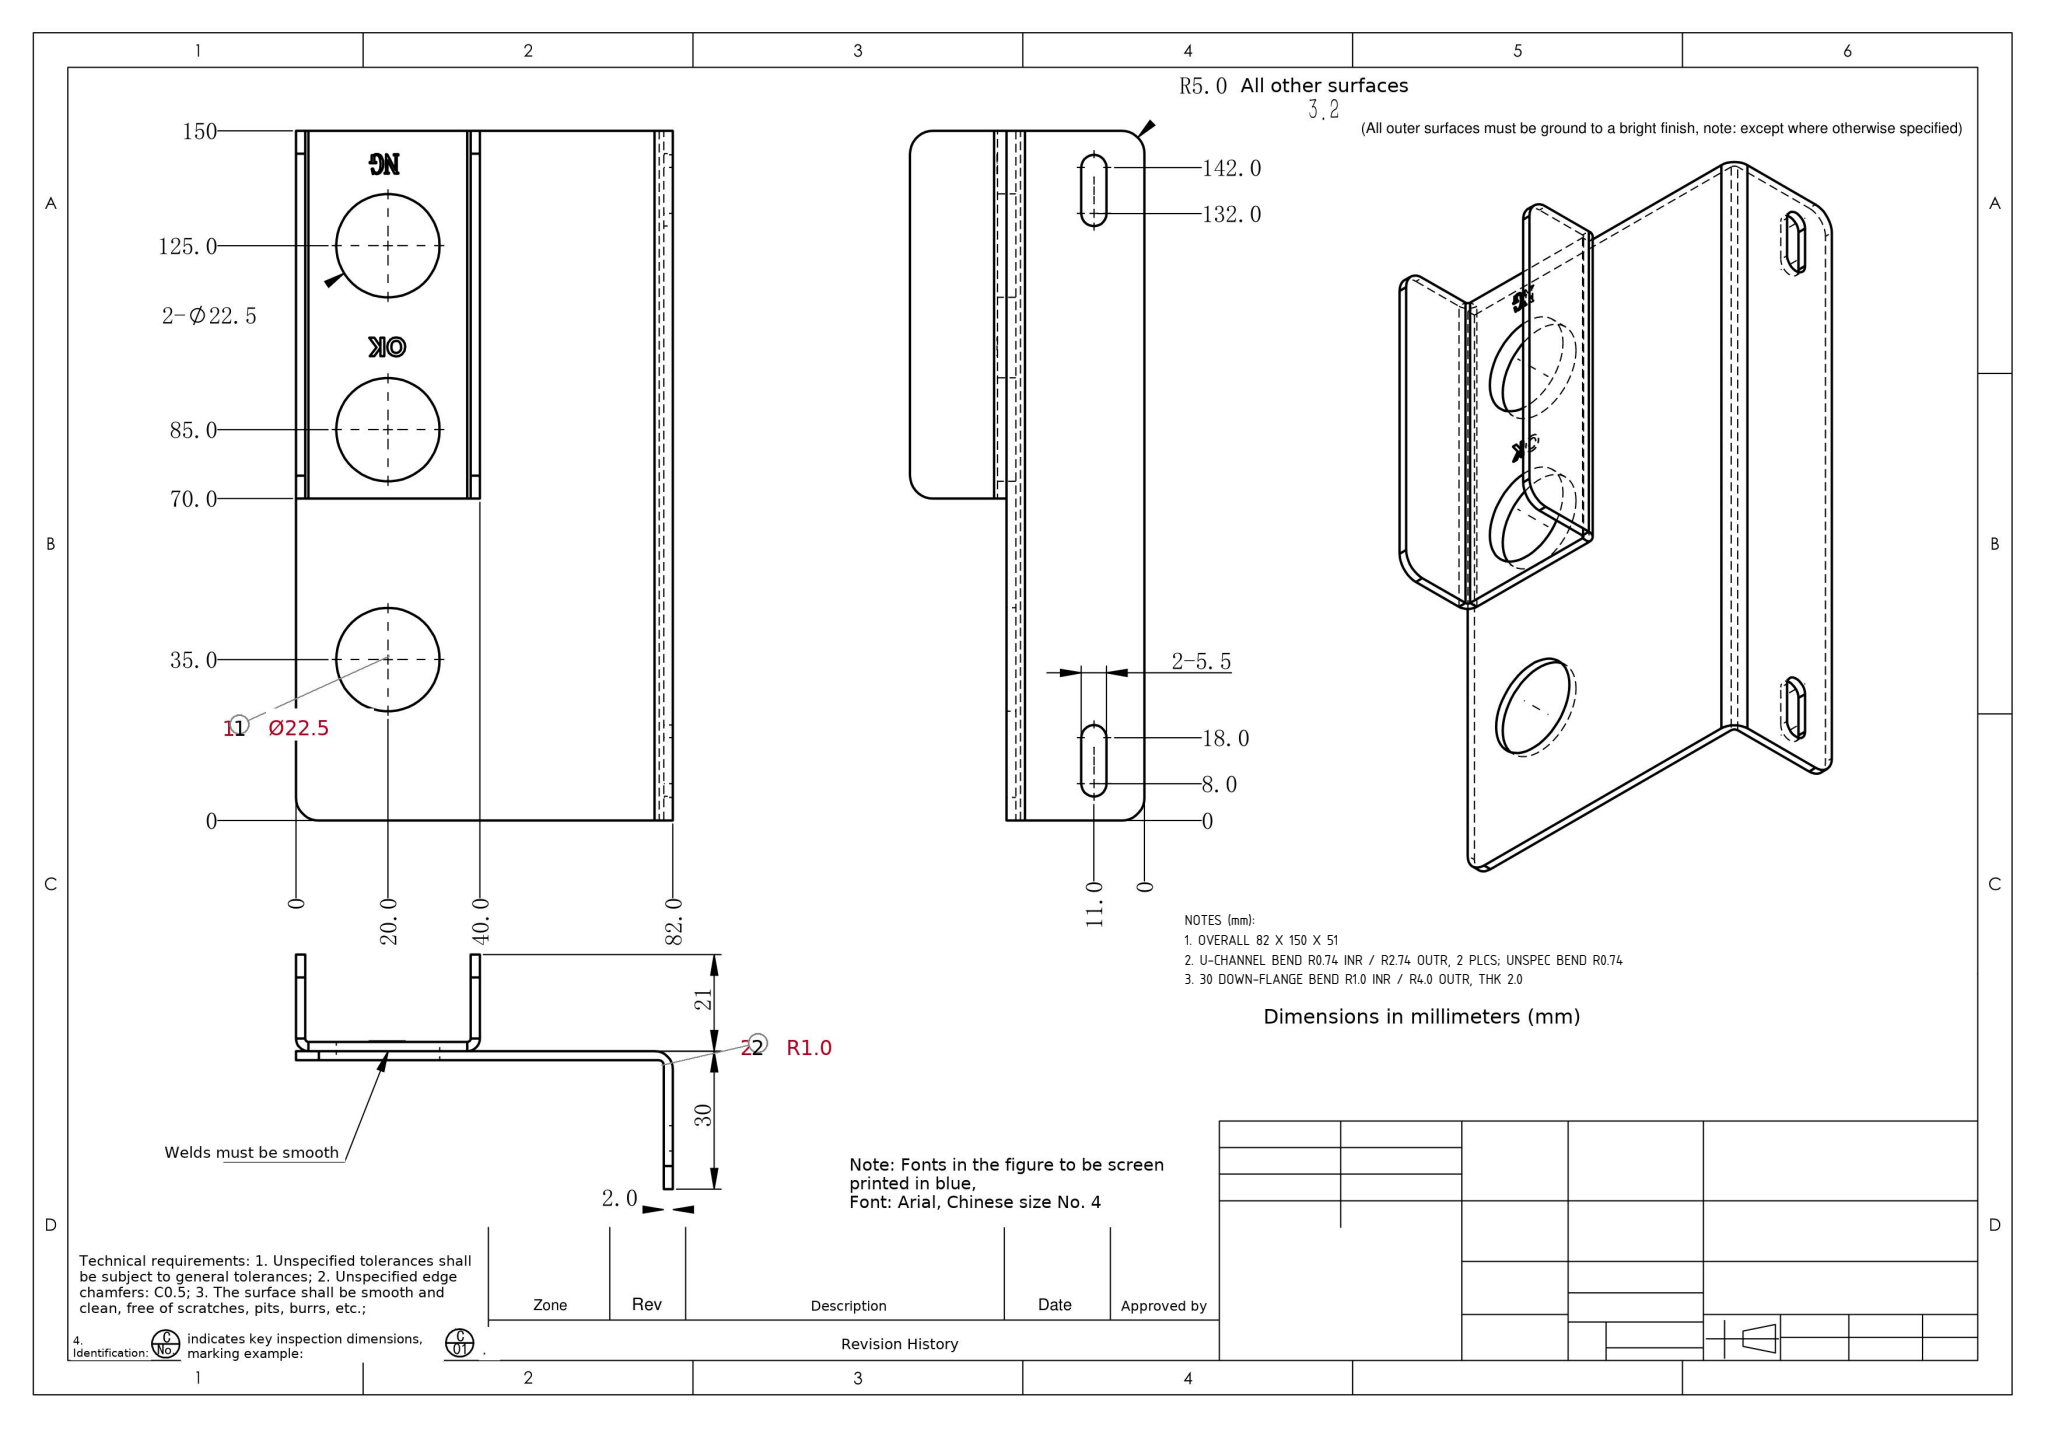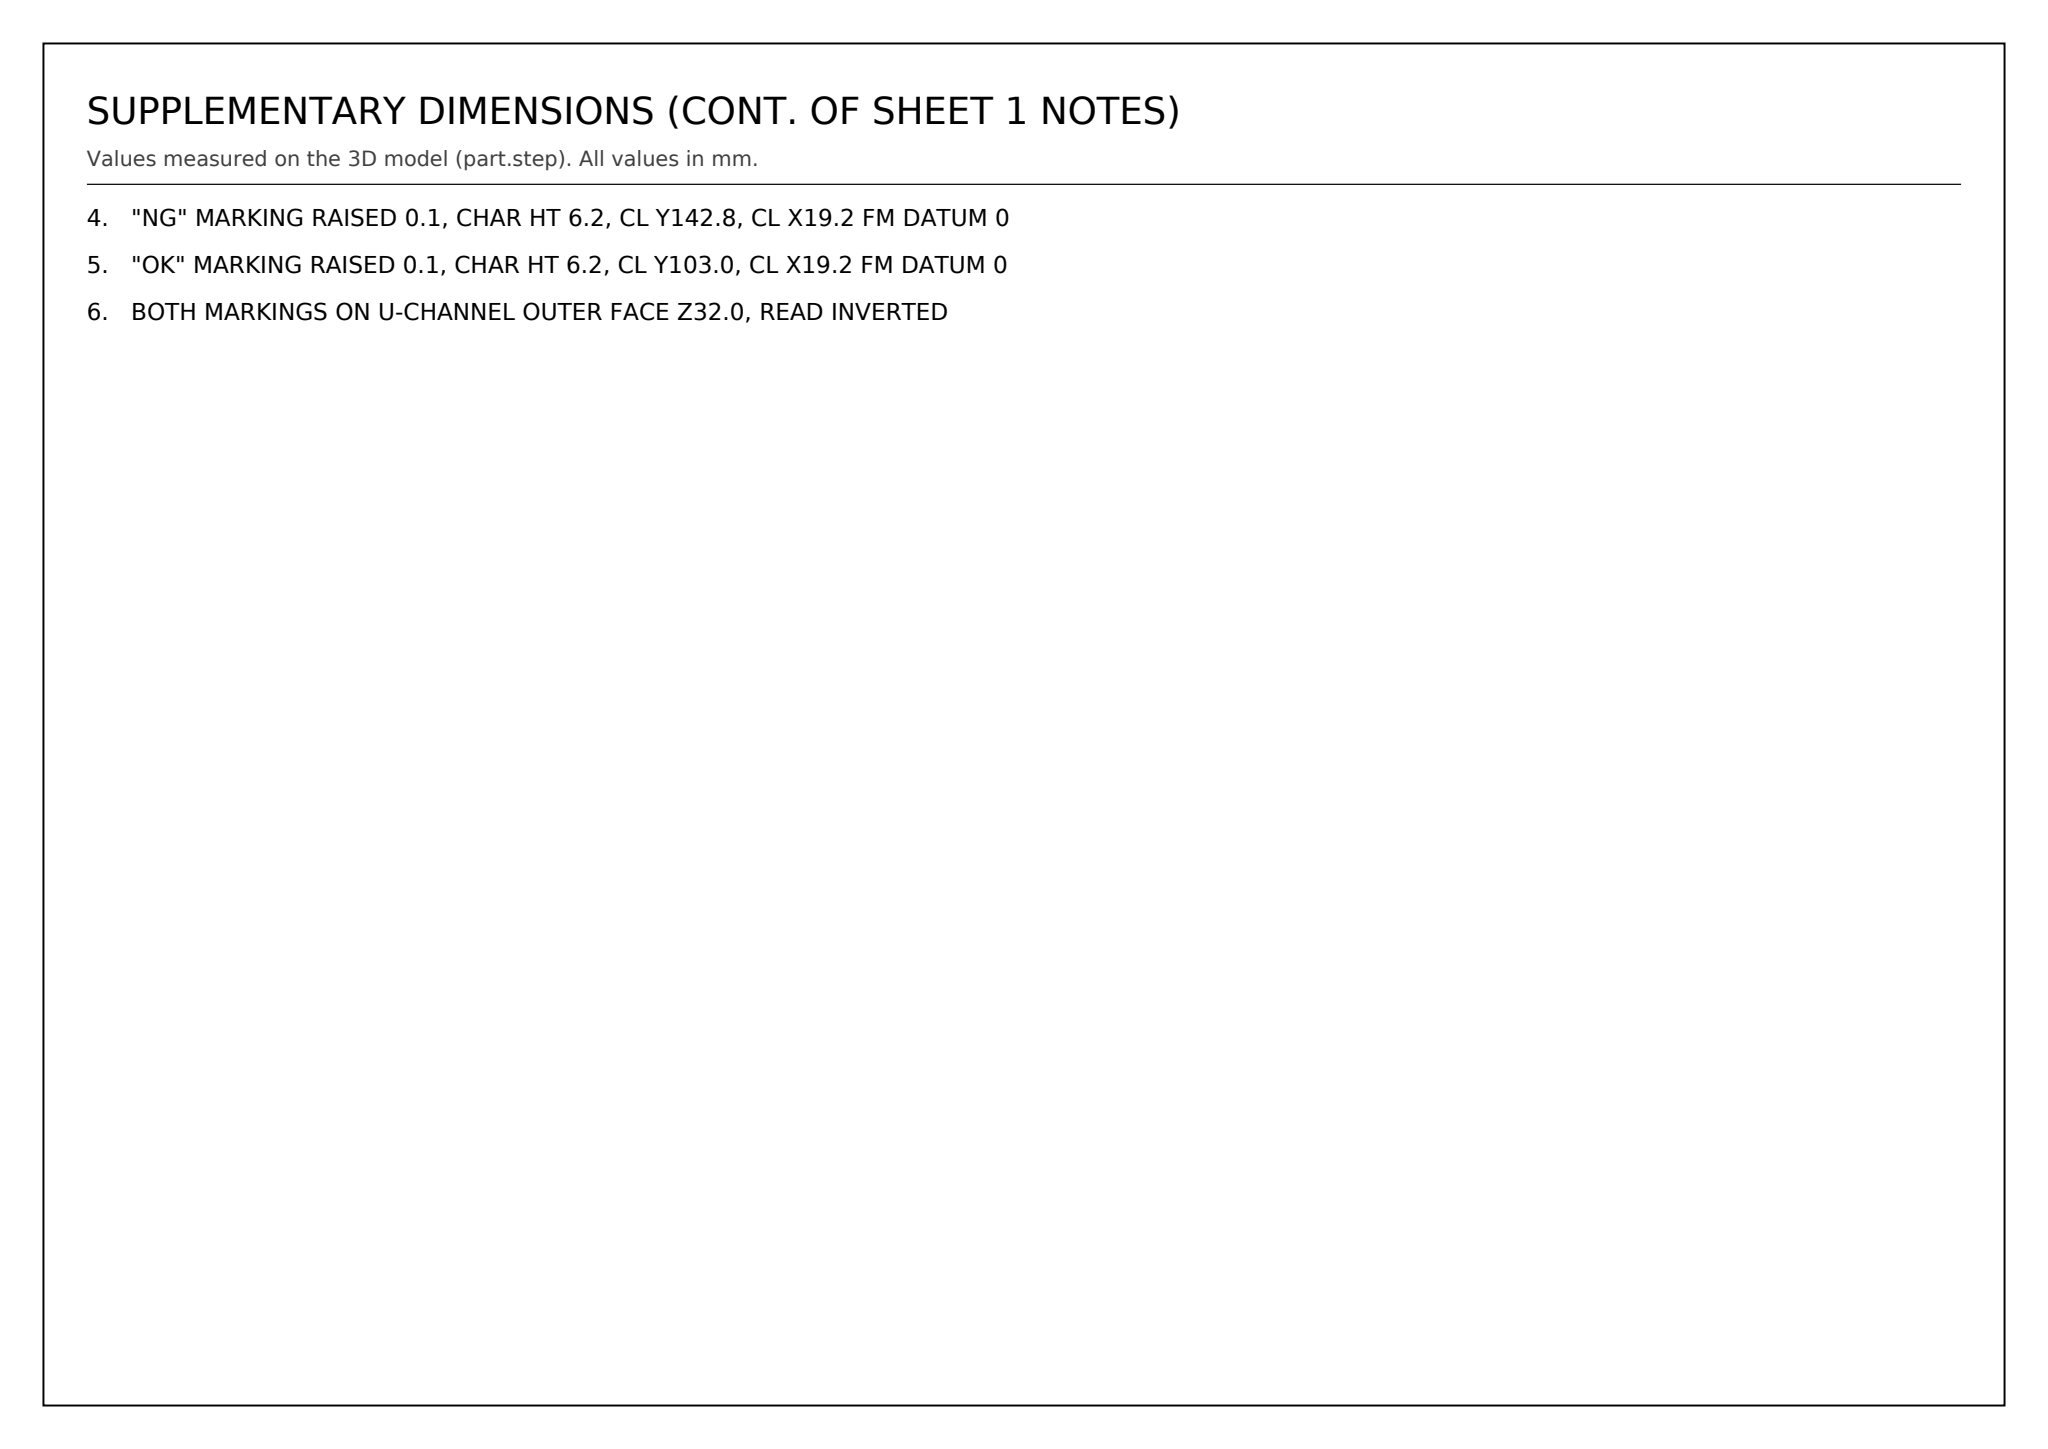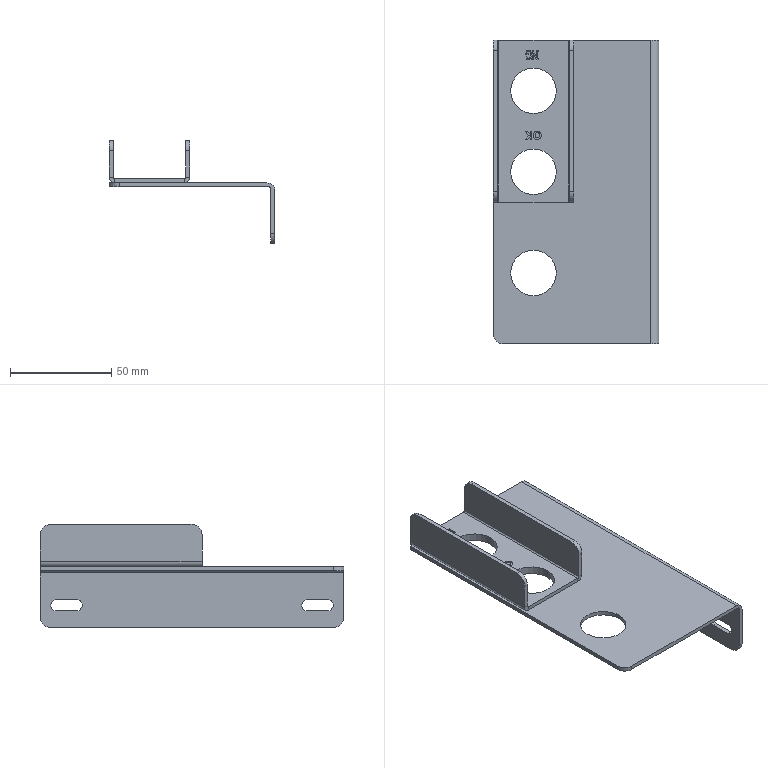Part | SolidWorks | mm | 1 solid | 129 faces | box 82 x 150 x 51 mm | volume 40395 mm3 | plane 76 | spline 28 | cylinder 25 | commonest cylinder face diameters 10 x7 22.5 x6 5.5 x6 5.473 x2 1.473 x2 8 x1 2 x1
Drawing notes:
OVERALL 82 X 150 X 51 | from the solid: bbox_xyz 82.0 x 150.0 x 51.0
U-CHANNEL BEND R0.74 INR / R2.74 OUTR, 2 PLCS; UNSPEC BEND R0.74 | from the solid: Cyl dia 1.473 (R0.737) & dia 5.473 (R2.737), axis Y, len 80, at (x2.74,z32.74) and (x37.26,z32.74) = inner+outer bend faces of channel legs
30 DOWN-FLANGE BEND R1.0 INR / R4.0 OUTR, THK 2.0 | from the solid: Cyl dia 2.0 axis Y len 150 at (x79.0,z27.0) = R1.0 inner; cyl dia 8.0 axis Y len 150 at (x78.0,z26.0) = R4.0 outer; planes x80/x82 give 2.0 thk
"NG" MARKING RAISED 0.1, CHAR HT 6.2, CL Y142.8, CL X19.2 FM DATUM 0 | from the solid: z-planes 32.0 & 32.1 (raised 0.1); x-planes 16.06-22.28 (ctr 19.17, ht 6.22); y-planes 140.64-144.88 (ctr 142.76)
"OK" MARKING RAISED 0.1, CHAR HT 6.2, CL Y103.0, CL X19.2 FM DATUM 0 | from the solid: z-planes 32.0 & 32.1 (raised 0.1); x-planes 16.06-22.28 (ctr 19.17, ht 6.22); y-planes 100.99-105.0 (ctr 103.0)
BOTH MARKINGS ON U-CHANNEL OUTER FACE Z32.0, READ INVERTED | from the solid: text solids lie on z=32.0 face, extruded to z=32.1